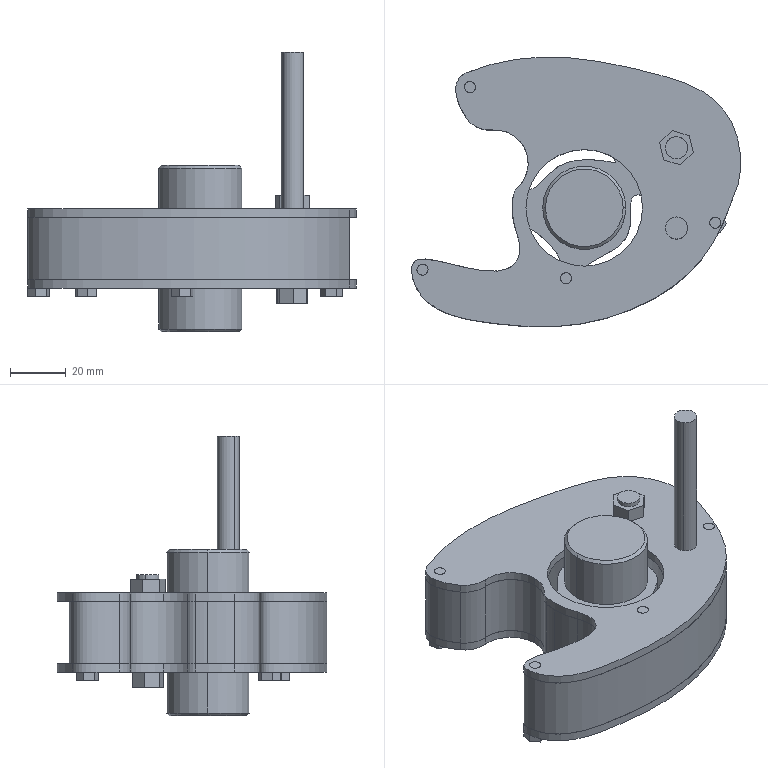Assembly | SolidWorks | mm | 15 component files | 25 solids | 437 faces | box 118.65 x 97.24 x 100.75 mm | volume 147593 mm3 | cylinder 207 | plane 126 | sphere 64 | spline 18 | torus 14 | cone 8 | commonest cylinder face diameters 4 x34 10.36 x32 6.643 x32 8 x23 4.02 x19 33.684 x15 24 x5 22 x4
Bill of materials:
10BoltSleeve-Length7.75 | 2 |  | Short thick-walled hollow cylinder (tube/sleeve shape) with a concentric through-bore and flat ends.
4Bolt | 4 |  | Hex-head bolt-like part: a thin hexagonal head with a long, plain cylindrical shank.
8Bolt35 | 1 |  | Hex-head bolt-like part with a thicker cylindrical shank and a taller hex head than the other hex-head shank parts.
8Bolt85 | 1 |  | Slender hex-head bolt- or pin-like part: a small, short hex head on a long, thin cylindrical shank.
8Nut | 1 |  | Hexagonal nut-like prism with a large central circular through-bore.
CenterAxis | 1 |  | Solid cylinder (pin/dowel-like) with small chamfers or edge breaks on both end edges.
ChainGuideSeat | 1 |  | Irregular curved, horn- or crescent-shaped plate-like body of constant thickness. It has a large central bore, several small and medium round holes, and lightening pockets that leave a perimeter rim and internal webs.
Gear-DragChain | 1 |  | Toothed ring resembling a sprocket or gear: roughly 15 rounded teeth around the outer edge, a large central bore, and a slightly recessed or stepped annular face next to the bore.
RollerBearing22_8Thickness7 | 1 |  | Ball-bearing-like annular body: an outer ring, an inner ring with a bore, and eight spherical rolling elements in the gap between them.
Sub-plate | 2 |  | Thin, flat plate with an irregular curved outline and two hooked arms. It has a large central circular hole, two medium holes, and several small holes, including holes near the arm tips.
Mates:
1. concentric | Gear-DragChain-1 face at (94.618, 134.462, 49.288) dir (0, 0, -1) r 11 | ChainGuideSeat-1 face at (94.618, 134.462, 54.288) dir (0, 0, -1) r 17.5
2. concentric | ChainGuideSeat-1 face at (108.623, 107.473, 54.288) dir (0, 0, -1) r 2 | 4Bolt-3 face at (108.623, 107.473, 57.288) dir (0, 0, -1) r 2
3. concentric | Gear-DragChain-1 face at (94.618, 134.462, 49.288) dir (0, 0, -1) r 11 | RollerBearing22_8Thickness7-1 face at (94.618, 134.462, 27.522) dir (0, 0, 1) r 4
4. concentric | 8Bolt35-1 face at (94.618, 134.462, 63.788) dir (0, 0, -1) r 4 | 10BoltSleeve-Length7.75-2 face at (94.618, 134.462, 39.538) dir (0, 0, -1) r 4
5. concentric | 10BoltSleeve-Length7.75-1 face at (94.618, 134.462, 54.288) dir (0, 0, -1) r 4 | 8Bolt35-1 face at (94.618, 134.462, 63.788) dir (0, 0, -1) r 4
6. concentric | 8Bolt35-1 face at (94.618, 134.462, 63.788) dir (0, 0, -1) r 4 | RollerBearing22_8Thickness7-1 face at (94.618, 134.462, 27.522) dir (0, 0, 1) r 4
7. concentric | ChainGuideSeat-1 face at (94.618, 105.469, 54.288) dir (0, 0, -1) r 4 | 8Bolt85-1 face at (94.618, 105.469, 113.788) dir (0, 0, -1) r 4
8. concentric | ChainGuideSeat-1 face at (3.13, 90.555, 54.288) dir (0, 0, -1) r 2 | Sub-plate-3 face at (3.13, 90.555, 54.288) dir (0, 0, 1) r 2
9. concentric | ChainGuideSeat-1 face at (108.623, 107.473, 54.288) dir (0, 0, -1) r 2 | Sub-plate-3 face at (108.623, 107.473, 54.288) dir (0, 0, 1) r 2
10. coincident | ChainGuideSeat-1 face at (61.422, 112.819, 54.288) dir (0, 0, 1) | Sub-plate-3 face at (39.778, 70.114, 54.288) dir (0, 0, -1)
11. concentric | 4Bolt-3 face at (108.623, 107.473, 57.288) dir (0, 0, -1) r 2 | Sub-plate-4 face at (108.623, 107.473, 28.788) dir (0, 0, 1) r 2
12. concentric | ChainGuideSeat-1 face at (20.233, 156.314, 54.288) dir (0, 0, -1) r 2 | Sub-plate-4 face at (20.233, 156.314, 28.788) dir (0, 0, 1) r 2
13. coincident | ChainGuideSeat-1 face at (61.422, 112.819, 31.788) dir (0, 0, -1) | Sub-plate-4 face at (39.778, 70.114, 31.788) dir (0, 0, 1)
14. concentric | 4Bolt-1 face at (20.233, 156.314, 57.288) dir (0, 0, -1) r 2 | Sub-plate-4 face at (20.233, 156.314, 28.788) dir (0, 0, 1) r 2
15. concentric | 4Bolt-2 face at (3.13, 90.555, 57.288) dir (0, 0, -1) r 2 | Sub-plate-4 face at (3.13, 90.555, 28.788) dir (0, 0, 1) r 2
16. concentric | 4Bolt-4 face at (54.861, 87.463, 57.288) dir (0, 0, -1) r 2 | Sub-plate-4 face at (54.861, 87.463, 28.788) dir (0, 0, 1) r 2
17. coincident | 4Bolt-4 face at (54.861, 87.463, 28.788) dir (0, 0, 1) | Sub-plate-4 face at (39.778, 70.114, 28.788) dir (0, 0, -1)
18. coincident | 4Bolt-2 face at (3.13, 90.555, 28.788) dir (0, 0, 1) | Sub-plate-4 face at (39.778, 70.114, 28.788) dir (0, 0, -1)
19. coincident | 4Bolt-1 face at (20.233, 156.314, 28.788) dir (0, 0, 1) | Sub-plate-4 face at (39.778, 70.114, 28.788) dir (0, 0, -1)
20. coincident | 8Bolt85-1 face at (94.618, 105.469, 28.788) dir (0, 0, 1) | Sub-plate-4 face at (39.778, 70.114, 28.788) dir (0, 0, -1)
21. concentric | 8Bolt35-1 face at (94.618, 134.462, 63.788) dir (0, 0, -1) r 4 | 8Nut-1 face at (94.618, 134.462, 62.288) dir (0, 0, -1) r 4
22. coincident | Sub-plate-3 face at (39.778, 70.114, 57.288) dir (0, 0, 1) | 8Nut-1 face at (94.618, 134.462, 57.288) dir (0, 0, -1)
23. concentric | ChainGuideSeat-1 face at (61.422, 112.819, 54.288) dir (0, 0, -1) r 15 | CenterAxis-1 face at (61.422, 112.819, 73.038) dir (0, 0, -1) r 15
24. width | Sub-plate-3 face at (39.778, 70.114, 57.288) dir (0, 0, 1) | Sub-plate-4 face at (39.778, 70.114, 28.788) dir (0, 0, -1) | CenterAxis-1 face at (61.422, 112.819, 13.038) dir (0, 0, -1) | CenterAxis-1 face at (61.422, 112.819, 73.038) dir (0, 0, 1)